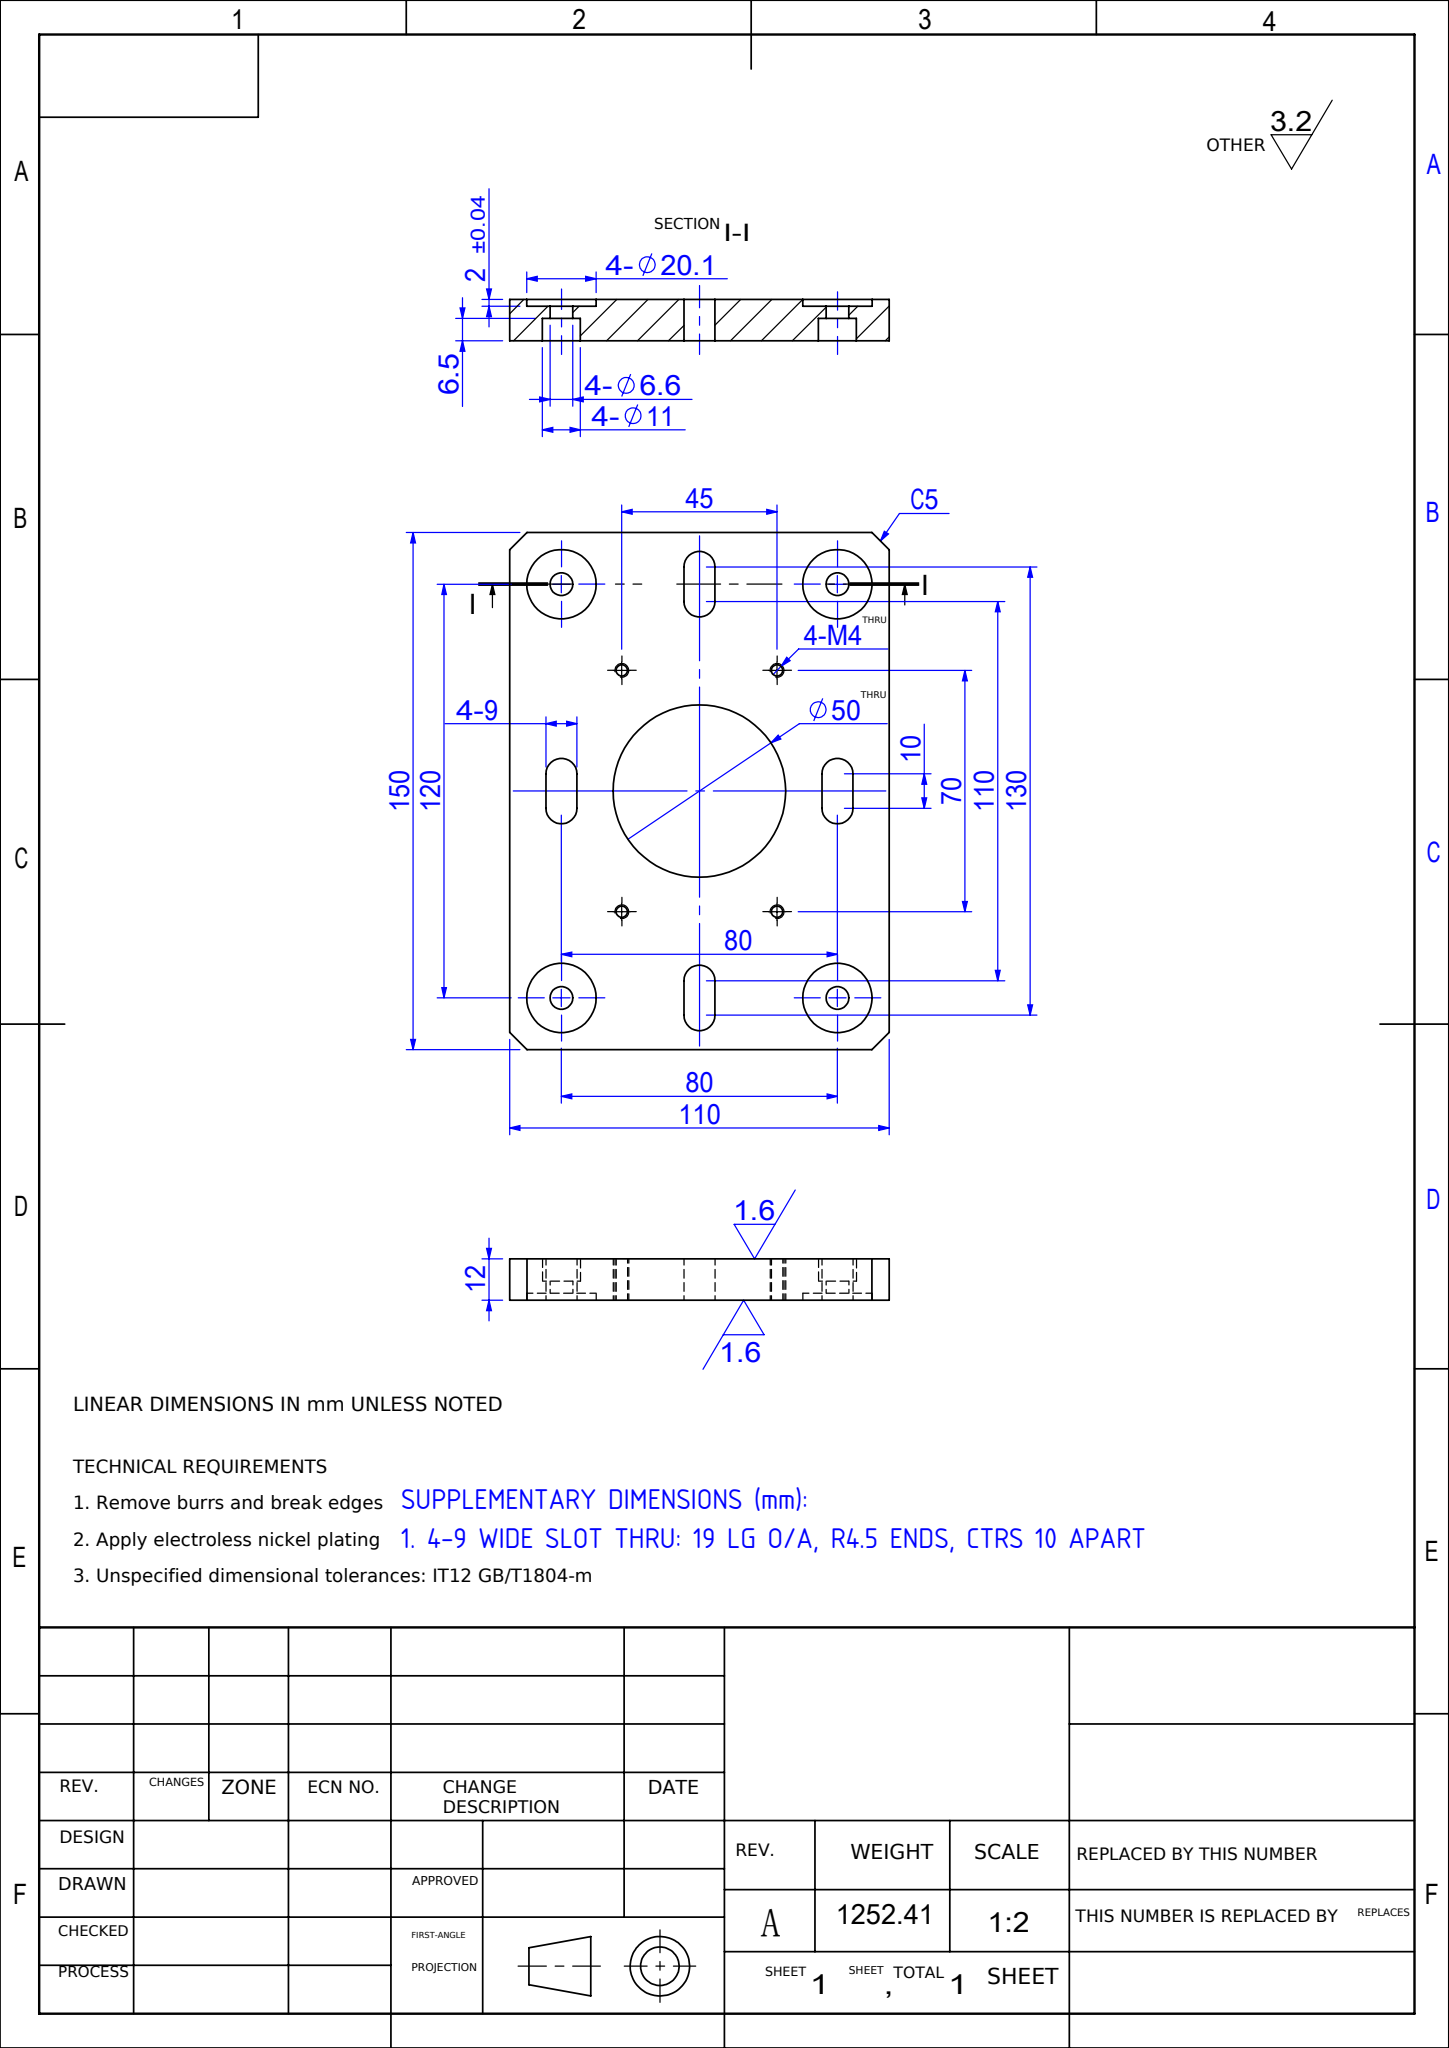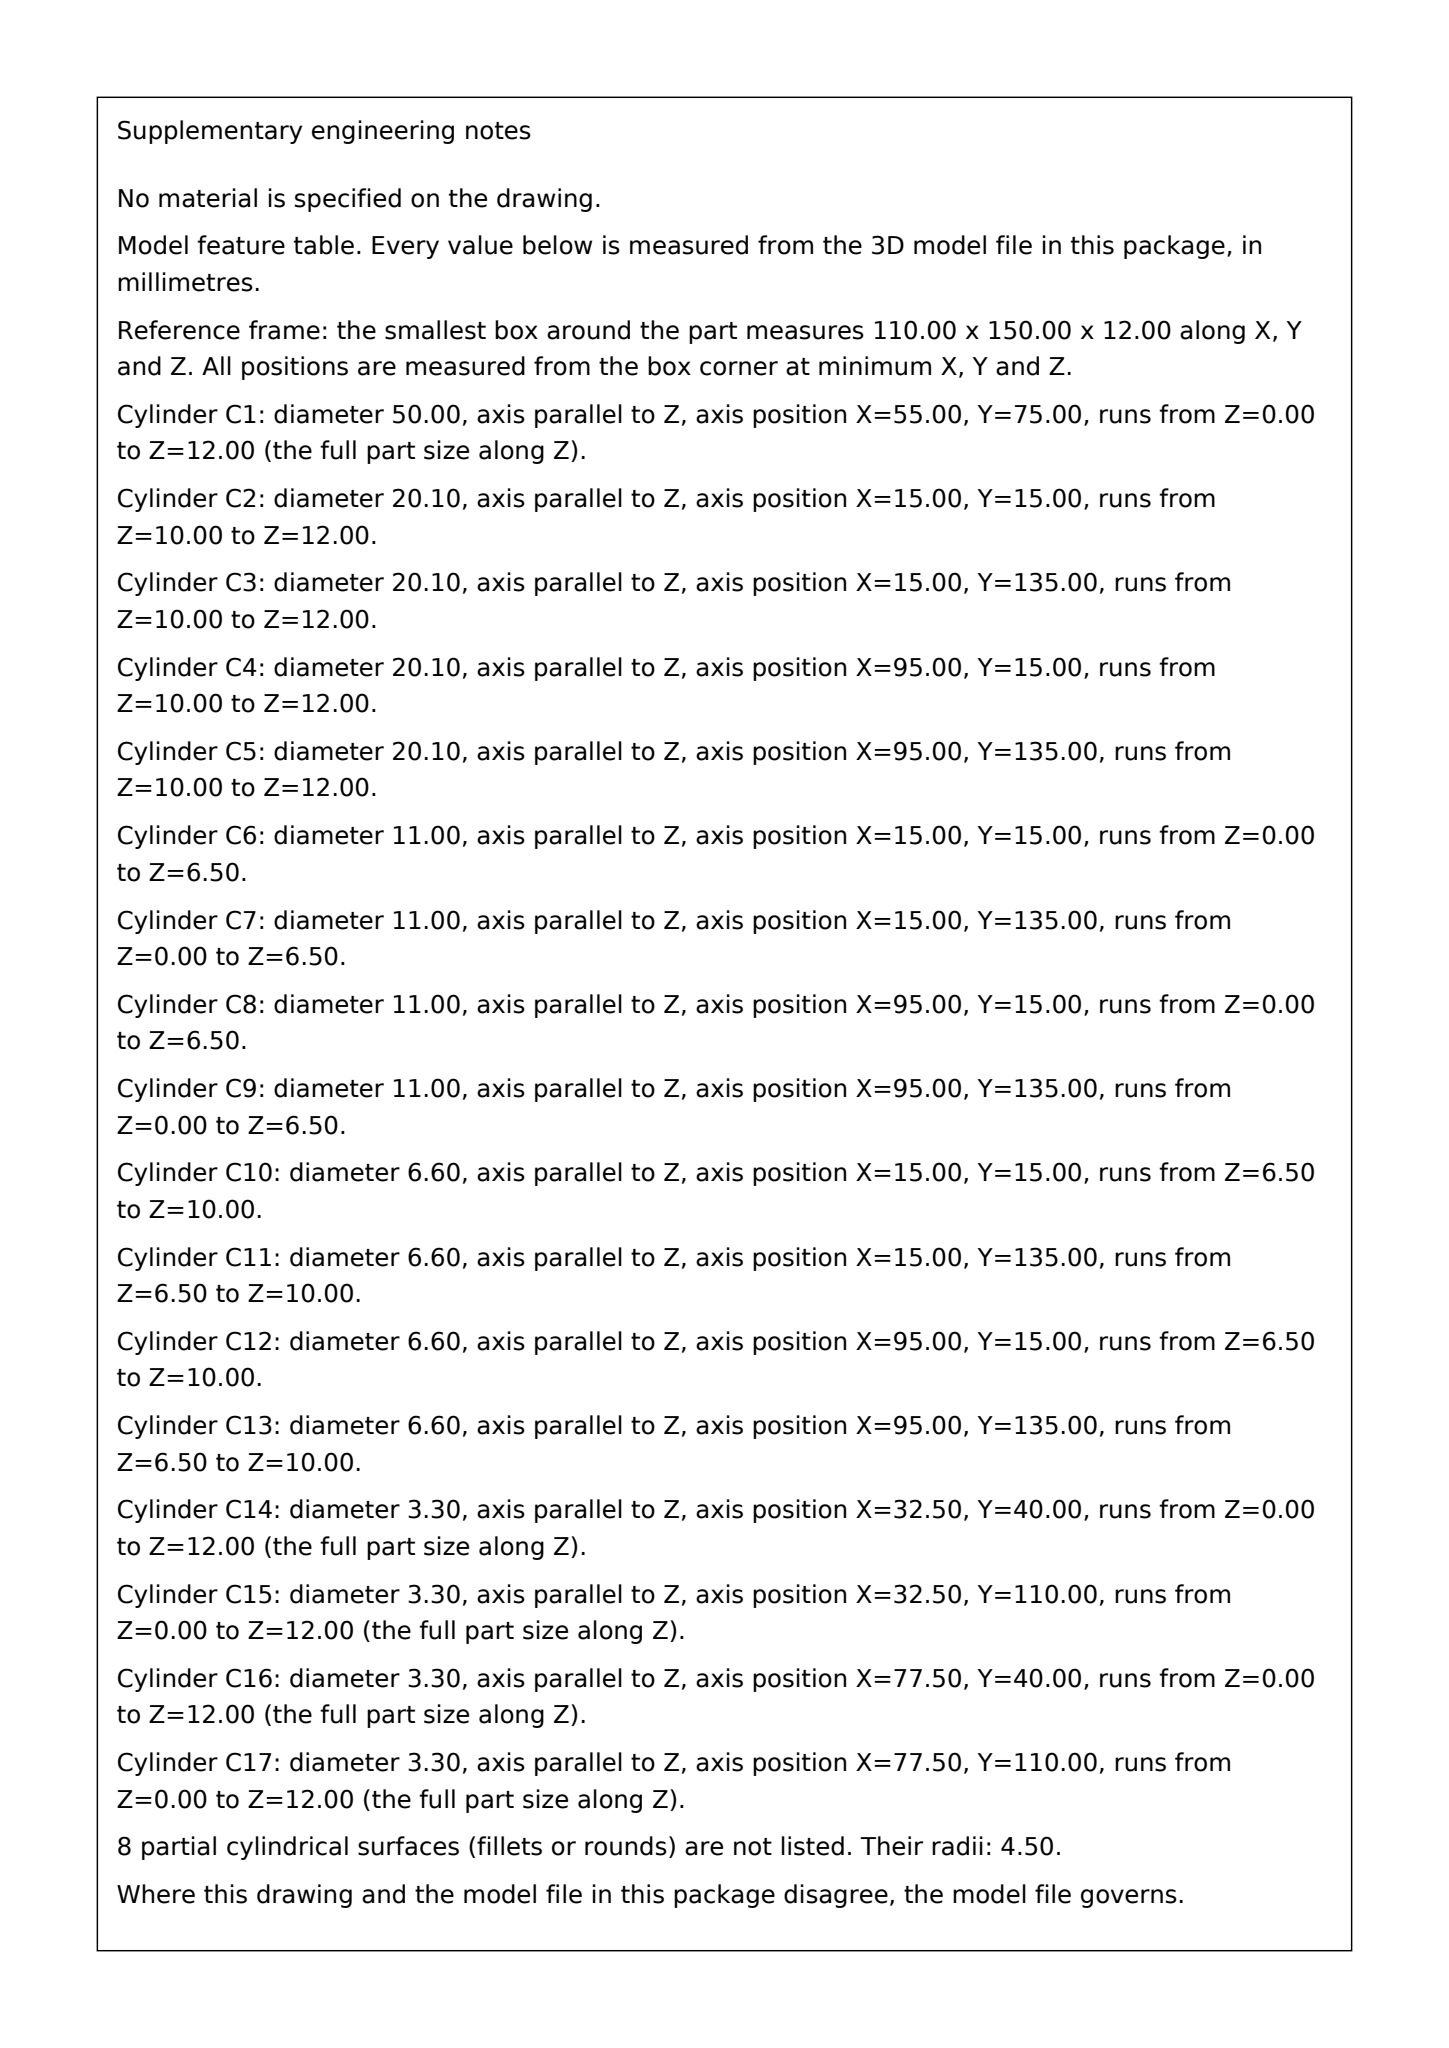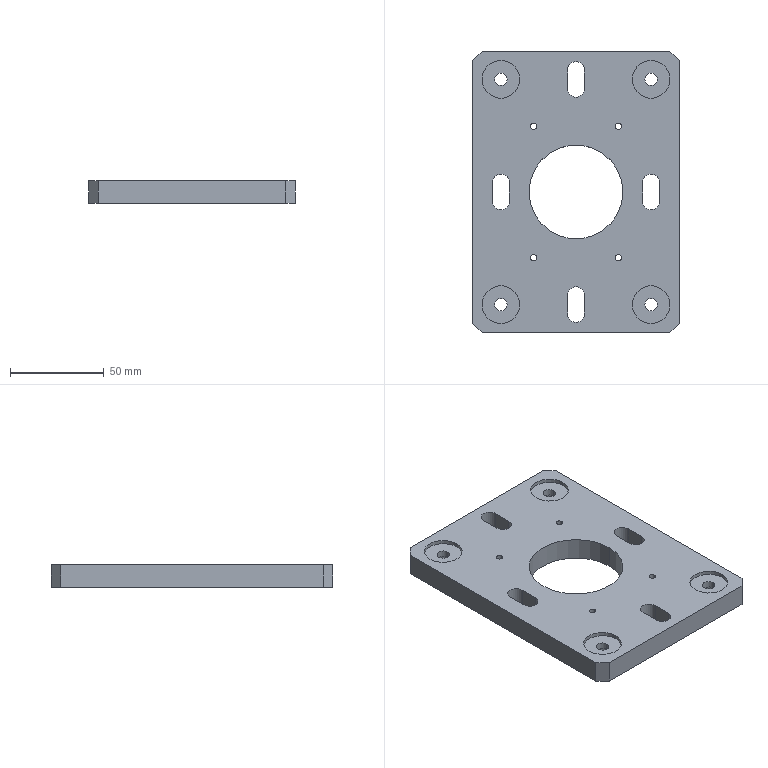Part | SolidWorks | mm | 1 solid | 68 faces | box 110 x 150 x 12 mm | volume 160566 mm3 | cylinder 42 | plane 26 | commonest cylinder face diameters 3.3 x8 20.1 x8 11 x8 6.6 x8 9 x8 50 x2
build123d program:
from build123d import *

# Parameters (mm, degrees)
SKETCH1_W                                       = 110
SKETCH1_H                                       = 150
EXTRUDE1_DEPTH                                  = 12
CUT_EXTRUDE1_DEPTH                              = 94.776
M6_HEX_SOCKET_HEAD_CAP_SCREW_CBORE1_D           = 6.6
M6_HEX_SOCKET_HEAD_CAP_SCREW_CBORE1_CBORE_D     = 11
M6_HEX_SOCKET_HEAD_CAP_SCREW_CBORE1_CBORE_DEPTH = 6.5
CHAMFER1_SIZE                                   = 5
SKETCH5_R                                       = 10.05
CUT_EXTRUDE2_DEPTH                              = 2
SKETCH6_R                                       = 25
CUT_EXTRUDE3_DEPTH                              = 94.776
M4_TAPPED_HOLE1_D                               = 3.3
MIRROR2_COPY_1_D                                = 3.3


with BuildPart() as part:
    # Sketch1 → Extrude1 (new body)
    with BuildSketch(Plane.XY):
        Rectangle(SKETCH1_W, SKETCH1_H)
    extrude(amount=EXTRUDE1_DEPTH)

    # Sketch2 → Cut-Extrude1 (cut, through all)
    with BuildSketch(Plane.XY.offset(12)):
        with BuildLine():
            Line((-35.5, 5), (-35.5, -5))
            ThreePointArc((-35.5, -5), (-40, -9.5), (-44.5, -5))
            Line((-44.5, -5), (-44.5, 5))
            ThreePointArc((-44.5, 5), (-40, 9.5), (-35.5, 5))
        make_face()
        with BuildLine():
            Line((-4.5, -65), (-4.5, -55))
            ThreePointArc((-4.5, -55), (0, -50.5), (4.5, -55))
            Line((4.5, -55), (4.5, -65))
            ThreePointArc((4.5, -65), (0, -69.5), (-4.5, -65))
        make_face()
        with BuildLine():
            Line((44.5, 5), (44.5, -5))
            ThreePointArc((44.5, -5), (40, -9.5), (35.5, -5))
            Line((35.5, -5), (35.5, 5))
            ThreePointArc((35.5, 5), (40, 9.5), (44.5, 5))
        make_face()
        with BuildLine():
            Line((4.5, 65), (4.5, 55))
            ThreePointArc((4.5, 55), (0, 50.5), (-4.5, 55))
            Line((-4.5, 55), (-4.5, 65))
            ThreePointArc((-4.5, 65), (0, 69.5), (4.5, 65))
        make_face()
    extrude(amount=-CUT_EXTRUDE1_DEPTH, mode=Mode.SUBTRACT)

    # M6 Hex Socket Head Cap Screw CBORE1 (through all)
    with Locations(Plane(origin=(0, 0, 0), x_dir=(-1, 0, 0), z_dir=(0, 0, -1))):
        with Locations((-40, -60), (40, 60), (-40, 60), (40, -60)):
            CounterBoreHole(M6_HEX_SOCKET_HEAD_CAP_SCREW_CBORE1_D / 2, M6_HEX_SOCKET_HEAD_CAP_SCREW_CBORE1_CBORE_D / 2, M6_HEX_SOCKET_HEAD_CAP_SCREW_CBORE1_CBORE_DEPTH)

    # Chamfer1
    chamfer1_edges = [part.edges().sort_by_distance(p)[0] for p in [
        (-55, 75, 6),
        (55, 75, 6),
        (55, -75, 6),
        (-55, -75, 6),
    ]]
    chamfer(chamfer1_edges, length=CHAMFER1_SIZE)

    # Sketch5 → Cut-Extrude2 (cut)
    with BuildSketch(Plane.XY.offset(12)):
        with Locations((-40, 60)):
            Circle(SKETCH5_R)
        with Locations((40, 60)):
            Circle(SKETCH5_R)
        with Locations((40, -60)):
            Circle(SKETCH5_R)
        with Locations((-40, -60)):
            Circle(SKETCH5_R)
    extrude(amount=-CUT_EXTRUDE2_DEPTH, mode=Mode.SUBTRACT)

    # Sketch6 → Cut-Extrude3 (cut, through all)
    with BuildSketch(Plane(origin=(0, 0, 0), x_dir=(-1, 0, 0), z_dir=(0, 0, -1))):
        Circle(SKETCH6_R)
    extrude(amount=-CUT_EXTRUDE3_DEPTH, mode=Mode.SUBTRACT)

    # M4 Tapped Hole1 (through all)
    with Locations(Plane(origin=(0, 0, 0), x_dir=(-1, 0, 0), z_dir=(0, 0, -1))):
        with Locations((22.5, 35)):
            m4_tapped_hole1 = Hole(M4_TAPPED_HOLE1_D / 2)

    # Mirror1: M4 Tapped Hole1 across plane
    add(m4_tapped_hole1.mirror(Plane.ZX), mode=Mode.SUBTRACT)

    # Mirror2: M4 Tapped Hole1 across plane
    add(m4_tapped_hole1.mirror(Plane(origin=(0, 0, 0), x_dir=(0, 0, 1), z_dir=(1, 0, 0))), mode=Mode.SUBTRACT)

    # Mirror2 copy 1 (through all)
    with Locations(Plane(origin=(0, 0, 0), x_dir=(1, 0, 0), z_dir=(0, 0, -1))):
        with Locations((22.5, 35)):
            Hole(MIRROR2_COPY_1_D / 2)


solid = part.part